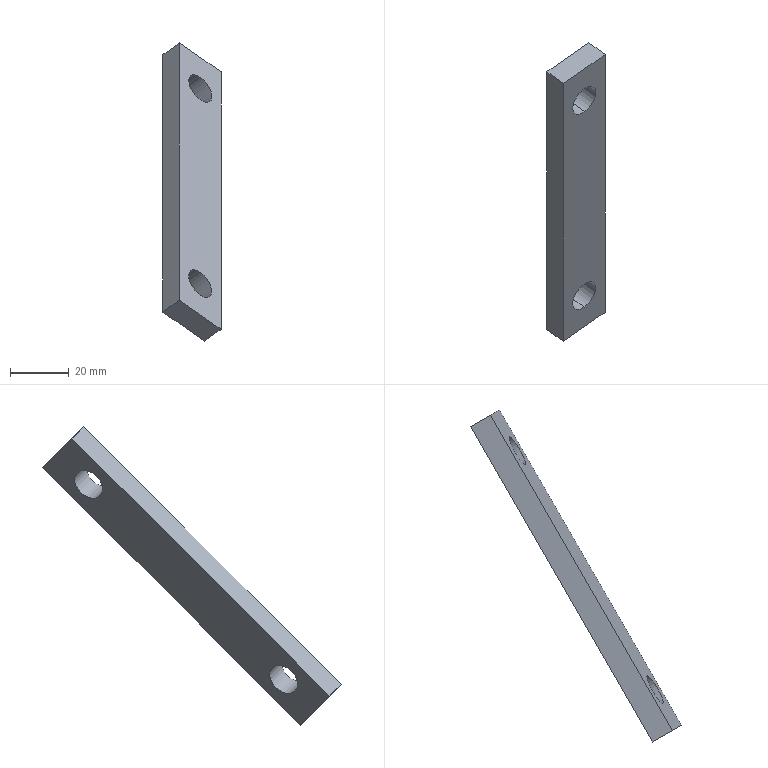Component | SolidWorks | SmallAxisAssembly-1_AdjustingRollerLowerPlate-1 | 1 solid | 10 faces | box 19.94 x 101.62 x 101.63 mm | volume 18319 mm3 | plane 6 | cylinder 4 | commonest cylinder face diameters 11 x4
build123d program:
from build123d import *

# Parameters (mm, degrees)
SKETCH1_W           = 124
SKETCH1_H           = 20
SKETCH1_R           = 5.5
BOSS_EXTRUDE1_DEPTH = 8


with BuildPart() as part:
    # Sketch1 → Boss-Extrude1 (new body)
    with BuildSketch(Plane.XY):
        Rectangle(SKETCH1_W, SKETCH1_H)
        with Locations((-47, 0)):
            Circle(SKETCH1_R, mode=Mode.SUBTRACT)
        with Locations((47, 0)):
            Circle(SKETCH1_R, mode=Mode.SUBTRACT)
    extrude(amount=BOSS_EXTRUDE1_DEPTH)


solid = part.part

# Placed as in the assembly
solid = solid.moved(Location((-6.727, 797.073, 252.085), (-134.971, -44.465, -89.958)))
STEP:
#1=COLOUR_RGB('',0.7922,0.8196,0.9333);
#2=FILL_AREA_STYLE_COLOUR('',#1);
#3=FILL_AREA_STYLE('',(#2));
#4=SURFACE_STYLE_FILL_AREA(#3);
#5=SURFACE_SIDE_STYLE('',(#4));
#6=SURFACE_STYLE_USAGE(.BOTH.,#5);
#7=PRESENTATION_STYLE_ASSIGNMENT((#6));
#8=CARTESIAN_POINT('',(-0.2657,30.226,8.769));
#9=VERTEX_POINT('',#8);
#10=CARTESIAN_POINT('',(-0.2659,29.919,8.463));
#11=VERTEX_POINT('',#10);
#12=CARTESIAN_POINT('',(-0.2658,30.072,8.616));
#13=DIRECTION('',(0.7005,-0.5049,0.5044));
#14=DIRECTION('',(-0.0005225,-0.7071,-0.7071));
#15=AXIS2_PLACEMENT_3D('',#12,#13,#14);
#16=CIRCLE('',#15,0.2165);
#17=EDGE_CURVE('',#9,#11,#16,.T.);
#18=ORIENTED_EDGE('',*,*,#17,.T.);
#19=CARTESIAN_POINT('',(-0.4866,30.078,8.304));
#20=VERTEX_POINT('',#19);
#21=CARTESIAN_POINT('',(-0.2659,29.919,8.463));
#22=DIRECTION('',(-0.7005,0.5049,-0.5044));
#23=VECTOR('',#22,39.37);
#24=LINE('',#21,#23);
#25=EDGE_CURVE('',#11,#20,#24,.T.);
#26=ORIENTED_EDGE('',*,*,#25,.T.);
#27=CARTESIAN_POINT('',(-0.4863,30.385,8.61));
#28=VERTEX_POINT('',#27);
#29=CARTESIAN_POINT('',(-0.4865,30.231,8.457));
#30=DIRECTION('',(0.7005,-0.5049,0.5044));
#31=DIRECTION('',(-0.0005225,-0.7071,-0.7071));
#32=AXIS2_PLACEMENT_3D('',#29,#30,#31);
#33=CIRCLE('',#32,0.2165);
#34=EDGE_CURVE('',#28,#20,#33,.T.);
#35=ORIENTED_EDGE('',*,*,#34,.F.);
#36=CARTESIAN_POINT('',(-0.2657,30.226,8.769));
#37=DIRECTION('',(-0.7005,0.5049,-0.5044));
#38=VECTOR('',#37,39.37);
#39=LINE('',#36,#38);
#40=EDGE_CURVE('',#9,#28,#39,.T.);
#41=ORIENTED_EDGE('',*,*,#40,.F.);
#42=EDGE_LOOP('',(#18,#26,#35,#41));
#43=FACE_OUTER_BOUND('',#42,.T.);
#44=CARTESIAN_POINT('',(-0.2658,30.072,8.616));
#45=DIRECTION('',(-0.7005,0.5049,-0.5044));
#46=DIRECTION('',(0.0005225,0.7071,0.7071));
#47=AXIS2_PLACEMENT_3D('',#44,#45,#46);
#48=CYLINDRICAL_SURFACE('',#47,0.2165);
#49=ADVANCED_FACE('',(#43),#48,.F.);
#50=CARTESIAN_POINT('',(-0.2638,32.842,11.386));
#51=VERTEX_POINT('',#50);
#52=CARTESIAN_POINT('',(-0.264,32.536,11.08));
#53=VERTEX_POINT('',#52);
#54=CARTESIAN_POINT('',(-0.2639,32.689,11.233));
#55=DIRECTION('',(0.7005,-0.5049,0.5044));
#56=DIRECTION('',(-0.0005225,-0.7071,-0.7071));
#57=AXIS2_PLACEMENT_3D('',#54,#55,#56);
#58=CIRCLE('',#57,0.2165);
#59=EDGE_CURVE('',#51,#53,#58,.T.);
#60=ORIENTED_EDGE('',*,*,#59,.T.);
#61=CARTESIAN_POINT('',(-0.4846,32.695,10.921));
#62=VERTEX_POINT('',#61);
#63=CARTESIAN_POINT('',(-0.264,32.536,11.08));
#64=DIRECTION('',(-0.7005,0.5049,-0.5044));
#65=VECTOR('',#64,39.37);
#66=LINE('',#63,#65);
#67=EDGE_CURVE('',#53,#62,#66,.T.);
#68=ORIENTED_EDGE('',*,*,#67,.T.);
#69=CARTESIAN_POINT('',(-0.4844,33.001,11.227));
#70=VERTEX_POINT('',#69);
#71=CARTESIAN_POINT('',(-0.4845,32.848,11.074));
#72=DIRECTION('',(0.7005,-0.5049,0.5044));
#73=DIRECTION('',(-0.0005225,-0.7071,-0.7071));
#74=AXIS2_PLACEMENT_3D('',#71,#72,#73);
#75=CIRCLE('',#74,0.2165);
#76=EDGE_CURVE('',#70,#62,#75,.T.);
#77=ORIENTED_EDGE('',*,*,#76,.F.);
#78=CARTESIAN_POINT('',(-0.2638,32.842,11.386));
#79=DIRECTION('',(-0.7005,0.5049,-0.5044));
#80=VECTOR('',#79,39.37);
#81=LINE('',#78,#80);
#82=EDGE_CURVE('',#51,#70,#81,.T.);
#83=ORIENTED_EDGE('',*,*,#82,.F.);
#84=EDGE_LOOP('',(#60,#68,#77,#83));
#85=FACE_OUTER_BOUND('',#84,.T.);
#86=CARTESIAN_POINT('',(-0.2639,32.689,11.233));
#87=DIRECTION('',(-0.7005,0.5049,-0.5044));
#88=DIRECTION('',(0.0005225,0.7071,0.7071));
#89=AXIS2_PLACEMENT_3D('',#86,#87,#88);
#90=CYLINDRICAL_SURFACE('',#89,0.2165);
#91=ADVANCED_FACE('',(#85),#90,.F.);
#92=CARTESIAN_POINT('',(-0.5471,29.46,8.394));
#93=VERTEX_POINT('',#92);
#94=CARTESIAN_POINT('',(0.01484,29.85,8.004));
#95=VERTEX_POINT('',#94);
#96=CARTESIAN_POINT('',(-0.5471,29.46,8.394));
#97=DIRECTION('',(0.7137,0.495,-0.4956));
#98=VECTOR('',#97,39.37);
#99=LINE('',#96,#98);
#100=EDGE_CURVE('',#93,#95,#99,.T.);
#101=ORIENTED_EDGE('',*,*,#100,.T.);
#102=CARTESIAN_POINT('',(0.01739,33.302,11.456));
#103=VERTEX_POINT('',#102);
#104=CARTESIAN_POINT('',(0.01739,33.302,11.456));
#105=DIRECTION('',(0.0005225,0.7071,0.7071));
#106=VECTOR('',#105,39.37);
#107=LINE('',#104,#106);
#108=EDGE_CURVE('',#95,#103,#107,.T.);
#109=ORIENTED_EDGE('',*,*,#108,.T.);
#110=CARTESIAN_POINT('',(-0.5446,32.912,11.846));
#111=VERTEX_POINT('',#110);
#112=CARTESIAN_POINT('',(-0.5446,32.912,11.846));
#113=DIRECTION('',(-0.7137,-0.495,0.4956));
#114=VECTOR('',#113,39.37);
#115=LINE('',#112,#114);
#116=EDGE_CURVE('',#103,#111,#115,.T.);
#117=ORIENTED_EDGE('',*,*,#116,.T.);
#118=CARTESIAN_POINT('',(-0.5446,32.912,11.846));
#119=DIRECTION('',(-0.0005225,-0.7071,-0.7071));
#120=VECTOR('',#119,39.37);
#121=LINE('',#118,#120);
#122=EDGE_CURVE('',#111,#93,#121,.T.);
#123=ORIENTED_EDGE('',*,*,#122,.T.);
#124=EDGE_LOOP('',(#101,#109,#117,#123));
#125=FACE_OUTER_BOUND('',#124,.T.);
#126=ORIENTED_EDGE('',*,*,#59,.F.);
#127=CARTESIAN_POINT('',(-0.2639,32.689,11.233));
#128=DIRECTION('',(0.7005,-0.5049,0.5044));
#129=DIRECTION('',(-0.0005225,-0.7071,-0.7071));
#130=AXIS2_PLACEMENT_3D('',#127,#128,#129);
#131=CIRCLE('',#130,0.2165);
#132=EDGE_CURVE('',#53,#51,#131,.T.);
#133=ORIENTED_EDGE('',*,*,#132,.F.);
#134=EDGE_LOOP('',(#126,#133));
#135=FACE_BOUND('',#134,.T.);
#136=ORIENTED_EDGE('',*,*,#17,.F.);
#137=CARTESIAN_POINT('',(-0.2658,30.072,8.616));
#138=DIRECTION('',(0.7005,-0.5049,0.5044));
#139=DIRECTION('',(-0.0005225,-0.7071,-0.7071));
#140=AXIS2_PLACEMENT_3D('',#137,#138,#139);
#141=CIRCLE('',#140,0.2165);
#142=EDGE_CURVE('',#11,#9,#141,.T.);
#143=ORIENTED_EDGE('',*,*,#142,.F.);
#144=EDGE_LOOP('',(#136,#143));
#145=FACE_BOUND('',#144,.T.);
#146=CARTESIAN_POINT('',(-0.2649,31.381,9.925));
#147=DIRECTION('',(-0.7005,0.5049,-0.5044));
#148=DIRECTION('',(0.0005225,0.7071,0.7071));
#149=AXIS2_PLACEMENT_3D('',#146,#147,#148);
#150=PLANE('',#149);
#151=ADVANCED_FACE('',(#125,#135,#145),#150,.F.);
#152=ORIENTED_EDGE('',*,*,#76,.T.);
#153=CARTESIAN_POINT('',(-0.4845,32.848,11.074));
#154=DIRECTION('',(0.7005,-0.5049,0.5044));
#155=DIRECTION('',(-0.0005225,-0.7071,-0.7071));
#156=AXIS2_PLACEMENT_3D('',#153,#154,#155);
#157=CIRCLE('',#156,0.2165);
#158=EDGE_CURVE('',#62,#70,#157,.T.);
#159=ORIENTED_EDGE('',*,*,#158,.T.);
#160=EDGE_LOOP('',(#152,#159));
#161=FACE_BOUND('',#160,.T.);
#162=CARTESIAN_POINT('',(-0.7677,29.619,8.235));
#163=VERTEX_POINT('',#162);
#164=CARTESIAN_POINT('',(-0.2058,30.009,7.845));
#165=VERTEX_POINT('',#164);
#166=CARTESIAN_POINT('',(-0.7677,29.619,8.235));
#167=DIRECTION('',(0.7137,0.495,-0.4956));
#168=VECTOR('',#167,39.37);
#169=LINE('',#166,#168);
#170=EDGE_CURVE('',#163,#165,#169,.T.);
#171=ORIENTED_EDGE('',*,*,#170,.F.);
#172=CARTESIAN_POINT('',(-0.7652,33.071,11.687));
#173=VERTEX_POINT('',#172);
#174=CARTESIAN_POINT('',(-0.7652,33.071,11.687));
#175=DIRECTION('',(-0.0005225,-0.7071,-0.7071));
#176=VECTOR('',#175,39.37);
#177=LINE('',#174,#176);
#178=EDGE_CURVE('',#173,#163,#177,.T.);
#179=ORIENTED_EDGE('',*,*,#178,.F.);
#180=CARTESIAN_POINT('',(-0.2032,33.461,11.297));
#181=VERTEX_POINT('',#180);
#182=CARTESIAN_POINT('',(-0.7652,33.071,11.687));
#183=DIRECTION('',(-0.7137,-0.495,0.4956));
#184=VECTOR('',#183,39.37);
#185=LINE('',#182,#184);
#186=EDGE_CURVE('',#181,#173,#185,.T.);
#187=ORIENTED_EDGE('',*,*,#186,.F.);
#188=CARTESIAN_POINT('',(-0.2032,33.461,11.297));
#189=DIRECTION('',(0.0005225,0.7071,0.7071));
#190=VECTOR('',#189,39.37);
#191=LINE('',#188,#190);
#192=EDGE_CURVE('',#165,#181,#191,.T.);
#193=ORIENTED_EDGE('',*,*,#192,.F.);
#194=EDGE_LOOP('',(#171,#179,#187,#193));
#195=FACE_OUTER_BOUND('',#194,.T.);
#196=ORIENTED_EDGE('',*,*,#34,.T.);
#197=CARTESIAN_POINT('',(-0.4865,30.231,8.457));
#198=DIRECTION('',(0.7005,-0.5049,0.5044));
#199=DIRECTION('',(-0.0005225,-0.7071,-0.7071));
#200=AXIS2_PLACEMENT_3D('',#197,#198,#199);
#201=CIRCLE('',#200,0.2165);
#202=EDGE_CURVE('',#20,#28,#201,.T.);
#203=ORIENTED_EDGE('',*,*,#202,.T.);
#204=EDGE_LOOP('',(#196,#203));
#205=FACE_BOUND('',#204,.T.);
#206=CARTESIAN_POINT('',(-0.4855,31.54,9.766));
#207=DIRECTION('',(-0.7005,0.5049,-0.5044));
#208=DIRECTION('',(0.0005225,0.7071,0.7071));
#209=AXIS2_PLACEMENT_3D('',#206,#207,#208);
#210=PLANE('',#209);
#211=ADVANCED_FACE('',(#161,#195,#205),#210,.T.);
#212=ORIENTED_EDGE('',*,*,#170,.T.);
#213=CARTESIAN_POINT('',(0.01484,29.85,8.004));
#214=DIRECTION('',(-0.7005,0.5049,-0.5044));
#215=VECTOR('',#214,39.37);
#216=LINE('',#213,#215);
#217=EDGE_CURVE('',#95,#165,#216,.T.);
#218=ORIENTED_EDGE('',*,*,#217,.F.);
#219=ORIENTED_EDGE('',*,*,#100,.F.);
#220=CARTESIAN_POINT('',(-0.5471,29.46,8.394));
#221=DIRECTION('',(-0.7005,0.5049,-0.5044));
#222=VECTOR('',#221,39.37);
#223=LINE('',#220,#222);
#224=EDGE_CURVE('',#93,#163,#223,.T.);
#225=ORIENTED_EDGE('',*,*,#224,.T.);
#226=EDGE_LOOP('',(#212,#218,#219,#225));
#227=FACE_OUTER_BOUND('',#226,.T.);
#228=CARTESIAN_POINT('',(-0.5471,29.46,8.394));
#229=DIRECTION('',(0.0005225,0.7071,0.7071));
#230=DIRECTION('',(0.7005,-0.5049,0.5044));
#231=AXIS2_PLACEMENT_3D('',#228,#229,#230);
#232=PLANE('',#231);
#233=ADVANCED_FACE('',(#227),#232,.F.);
#234=ORIENTED_EDGE('',*,*,#192,.T.);
#235=CARTESIAN_POINT('',(0.01739,33.302,11.456));
#236=DIRECTION('',(-0.7005,0.5049,-0.5044));
#237=VECTOR('',#236,39.37);
#238=LINE('',#235,#237);
#239=EDGE_CURVE('',#103,#181,#238,.T.);
#240=ORIENTED_EDGE('',*,*,#239,.F.);
#241=ORIENTED_EDGE('',*,*,#108,.F.);
#242=ORIENTED_EDGE('',*,*,#217,.T.);
#243=EDGE_LOOP('',(#234,#240,#241,#242));
#244=FACE_OUTER_BOUND('',#243,.T.);
#245=CARTESIAN_POINT('',(0.01739,33.302,11.456));
#246=DIRECTION('',(-0.7137,-0.495,0.4956));
#247=DIRECTION('',(-0.0005225,-0.7071,-0.7071));
#248=AXIS2_PLACEMENT_3D('',#245,#246,#247);
#249=PLANE('',#248);
#250=ADVANCED_FACE('',(#244),#249,.F.);
#251=ORIENTED_EDGE('',*,*,#186,.T.);
#252=CARTESIAN_POINT('',(-0.5446,32.912,11.846));
#253=DIRECTION('',(-0.7005,0.5049,-0.5044));
#254=VECTOR('',#253,39.37);
#255=LINE('',#252,#254);
#256=EDGE_CURVE('',#111,#173,#255,.T.);
#257=ORIENTED_EDGE('',*,*,#256,.F.);
#258=ORIENTED_EDGE('',*,*,#116,.F.);
#259=ORIENTED_EDGE('',*,*,#239,.T.);
#260=EDGE_LOOP('',(#251,#257,#258,#259));
#261=FACE_OUTER_BOUND('',#260,.T.);
#262=CARTESIAN_POINT('',(-0.5446,32.912,11.846));
#263=DIRECTION('',(-0.0005225,-0.7071,-0.7071));
#264=DIRECTION('',(-0.7005,0.5049,-0.5044));
#265=AXIS2_PLACEMENT_3D('',#262,#263,#264);
#266=PLANE('',#265);
#267=ADVANCED_FACE('',(#261),#266,.F.);
#268=ORIENTED_EDGE('',*,*,#178,.T.);
#269=ORIENTED_EDGE('',*,*,#224,.F.);
#270=ORIENTED_EDGE('',*,*,#122,.F.);
#271=ORIENTED_EDGE('',*,*,#256,.T.);
#272=EDGE_LOOP('',(#268,#269,#270,#271));
#273=FACE_OUTER_BOUND('',#272,.T.);
#274=CARTESIAN_POINT('',(-0.5446,32.912,11.846));
#275=DIRECTION('',(0.7137,0.495,-0.4956));
#276=DIRECTION('',(0.7005,-0.5049,0.5044));
#277=AXIS2_PLACEMENT_3D('',#274,#275,#276);
#278=PLANE('',#277);
#279=ADVANCED_FACE('',(#273),#278,.F.);
#280=ORIENTED_EDGE('',*,*,#67,.F.);
#281=ORIENTED_EDGE('',*,*,#132,.T.);
#282=ORIENTED_EDGE('',*,*,#82,.T.);
#283=ORIENTED_EDGE('',*,*,#158,.F.);
#284=EDGE_LOOP('',(#280,#281,#282,#283));
#285=FACE_OUTER_BOUND('',#284,.T.);
#286=CARTESIAN_POINT('',(-0.2639,32.689,11.233));
#287=DIRECTION('',(-0.7005,0.5049,-0.5044));
#288=DIRECTION('',(0.0005225,0.7071,0.7071));
#289=AXIS2_PLACEMENT_3D('',#286,#287,#288);
#290=CYLINDRICAL_SURFACE('',#289,0.2165);
#291=ADVANCED_FACE('',(#285),#290,.F.);
#292=ORIENTED_EDGE('',*,*,#25,.F.);
#293=ORIENTED_EDGE('',*,*,#142,.T.);
#294=ORIENTED_EDGE('',*,*,#40,.T.);
#295=ORIENTED_EDGE('',*,*,#202,.F.);
#296=EDGE_LOOP('',(#292,#293,#294,#295));
#297=FACE_OUTER_BOUND('',#296,.T.);
#298=CARTESIAN_POINT('',(-0.2658,30.072,8.616));
#299=DIRECTION('',(-0.7005,0.5049,-0.5044));
#300=DIRECTION('',(0.0005225,0.7071,0.7071));
#301=AXIS2_PLACEMENT_3D('',#298,#299,#300);
#302=CYLINDRICAL_SURFACE('',#301,0.2165);
#303=ADVANCED_FACE('',(#297),#302,.F.);
#304=CLOSED_SHELL('',(#49,#91,#151,#211,#233,#250,#267,#279,#291,#303));
#305=MANIFOLD_SOLID_BREP('',#304);
#306=STYLED_ITEM('',(#7),#305);
#307=(LENGTH_UNIT()NAMED_UNIT(*)SI_UNIT($,.METRE.));
#308=LENGTH_MEASURE_WITH_UNIT(LENGTH_MEASURE(0.0254),#307);
#309=DIMENSIONAL_EXPONENTS(1.,0.,0.,0.,0.,0.,0.);
#310=(CONVERSION_BASED_UNIT('',#308)LENGTH_UNIT()NAMED_UNIT(#309));
#311=UNCERTAINTY_MEASURE_WITH_UNIT(LENGTH_MEASURE(0.00001),#310,'','');
#312=(NAMED_UNIT(*)PLANE_ANGLE_UNIT()SI_UNIT($,.RADIAN.));
#313=(NAMED_UNIT(*)SI_UNIT($,.STERADIAN.)SOLID_ANGLE_UNIT());
#314=(GEOMETRIC_REPRESENTATION_CONTEXT(3)GLOBAL_UNCERTAINTY_ASSIGNED_CONTEXT((#311))GLOBAL_UNIT_ASSIGNED_CONTEXT((#310,#312,#313))REPRESENTATION_CONTEXT('',''));
#315=MECHANICAL_DESIGN_GEOMETRIC_PRESENTATION_REPRESENTATION('',(#306),#314);
#316=PRESENTATION_LAYER_ASSIGNMENT('','',(#306));
#317=CARTESIAN_POINT('',(0.,0.,0.));
#318=DIRECTION('',(0.,0.,1.));
#319=DIRECTION('',(1.,0.,0.));
#320=AXIS2_PLACEMENT_3D('',#317,#318,#319);
#321=(LENGTH_UNIT()NAMED_UNIT(*)SI_UNIT($,.METRE.));
#322=LENGTH_MEASURE_WITH_UNIT(LENGTH_MEASURE(0.0254),#321);
#323=DIMENSIONAL_EXPONENTS(1.,0.,0.,0.,0.,0.,0.);
#324=(CONVERSION_BASED_UNIT('',#322)LENGTH_UNIT()NAMED_UNIT(#323));
#325=UNCERTAINTY_MEASURE_WITH_UNIT(LENGTH_MEASURE(0.00001),#324,'','');
#326=(NAMED_UNIT(*)PLANE_ANGLE_UNIT()SI_UNIT($,.RADIAN.));
#327=(NAMED_UNIT(*)SI_UNIT($,.STERADIAN.)SOLID_ANGLE_UNIT());
#328=(GEOMETRIC_REPRESENTATION_CONTEXT(3)GLOBAL_UNCERTAINTY_ASSIGNED_CONTEXT((#325))GLOBAL_UNIT_ASSIGNED_CONTEXT((#324,#326,#327))REPRESENTATION_CONTEXT('',''));
#329=ADVANCED_BREP_SHAPE_REPRESENTATION('',(#305,#320),#328);